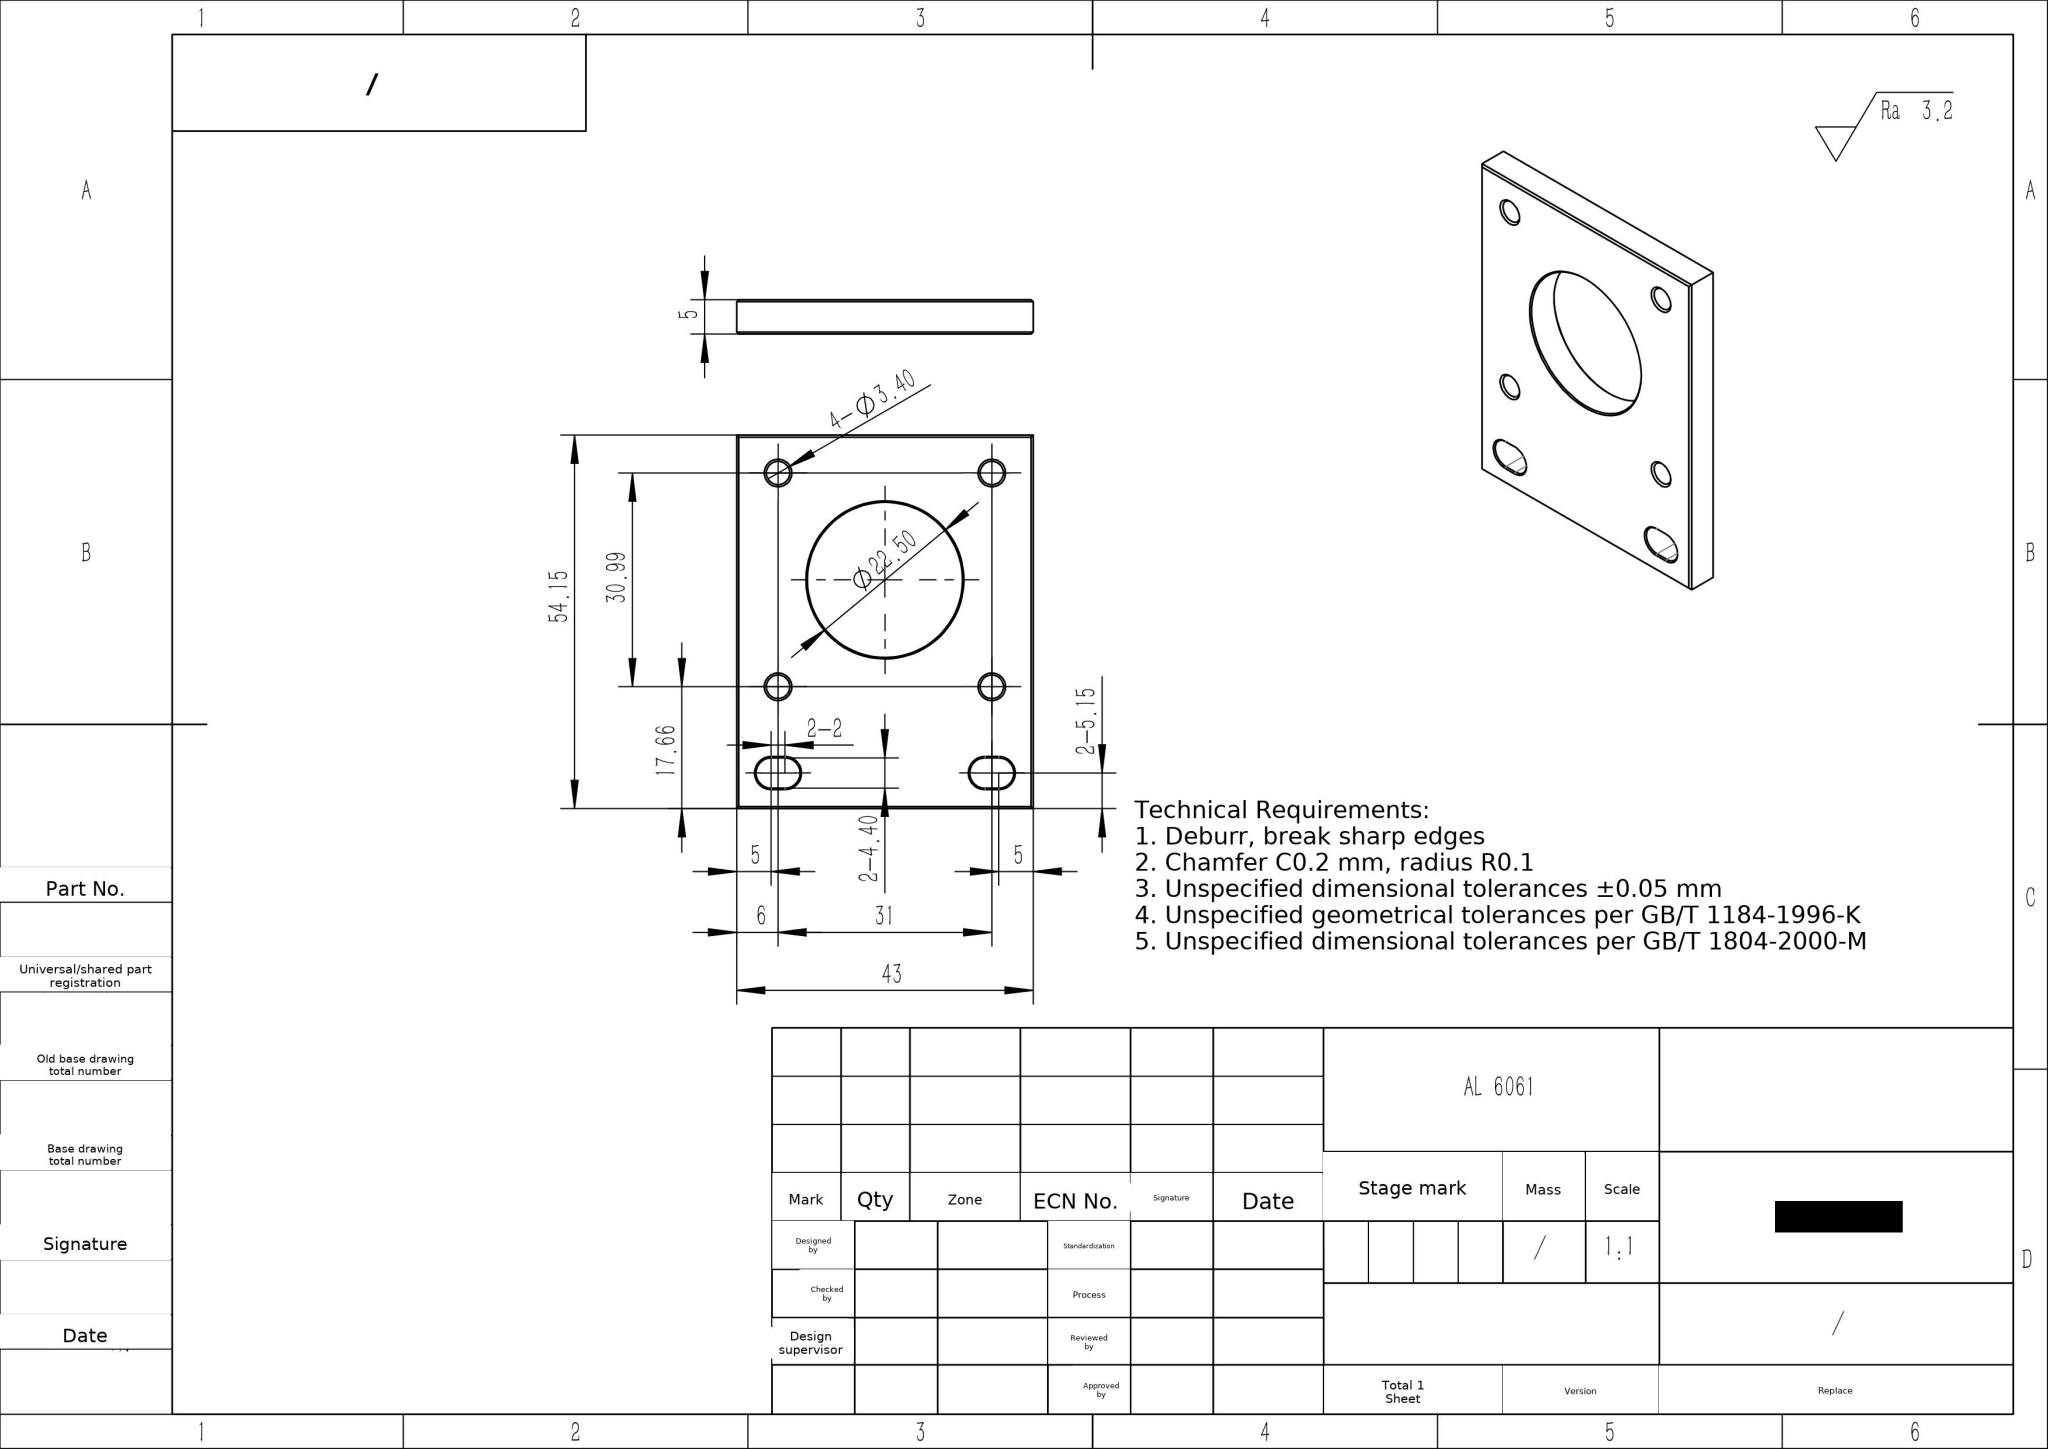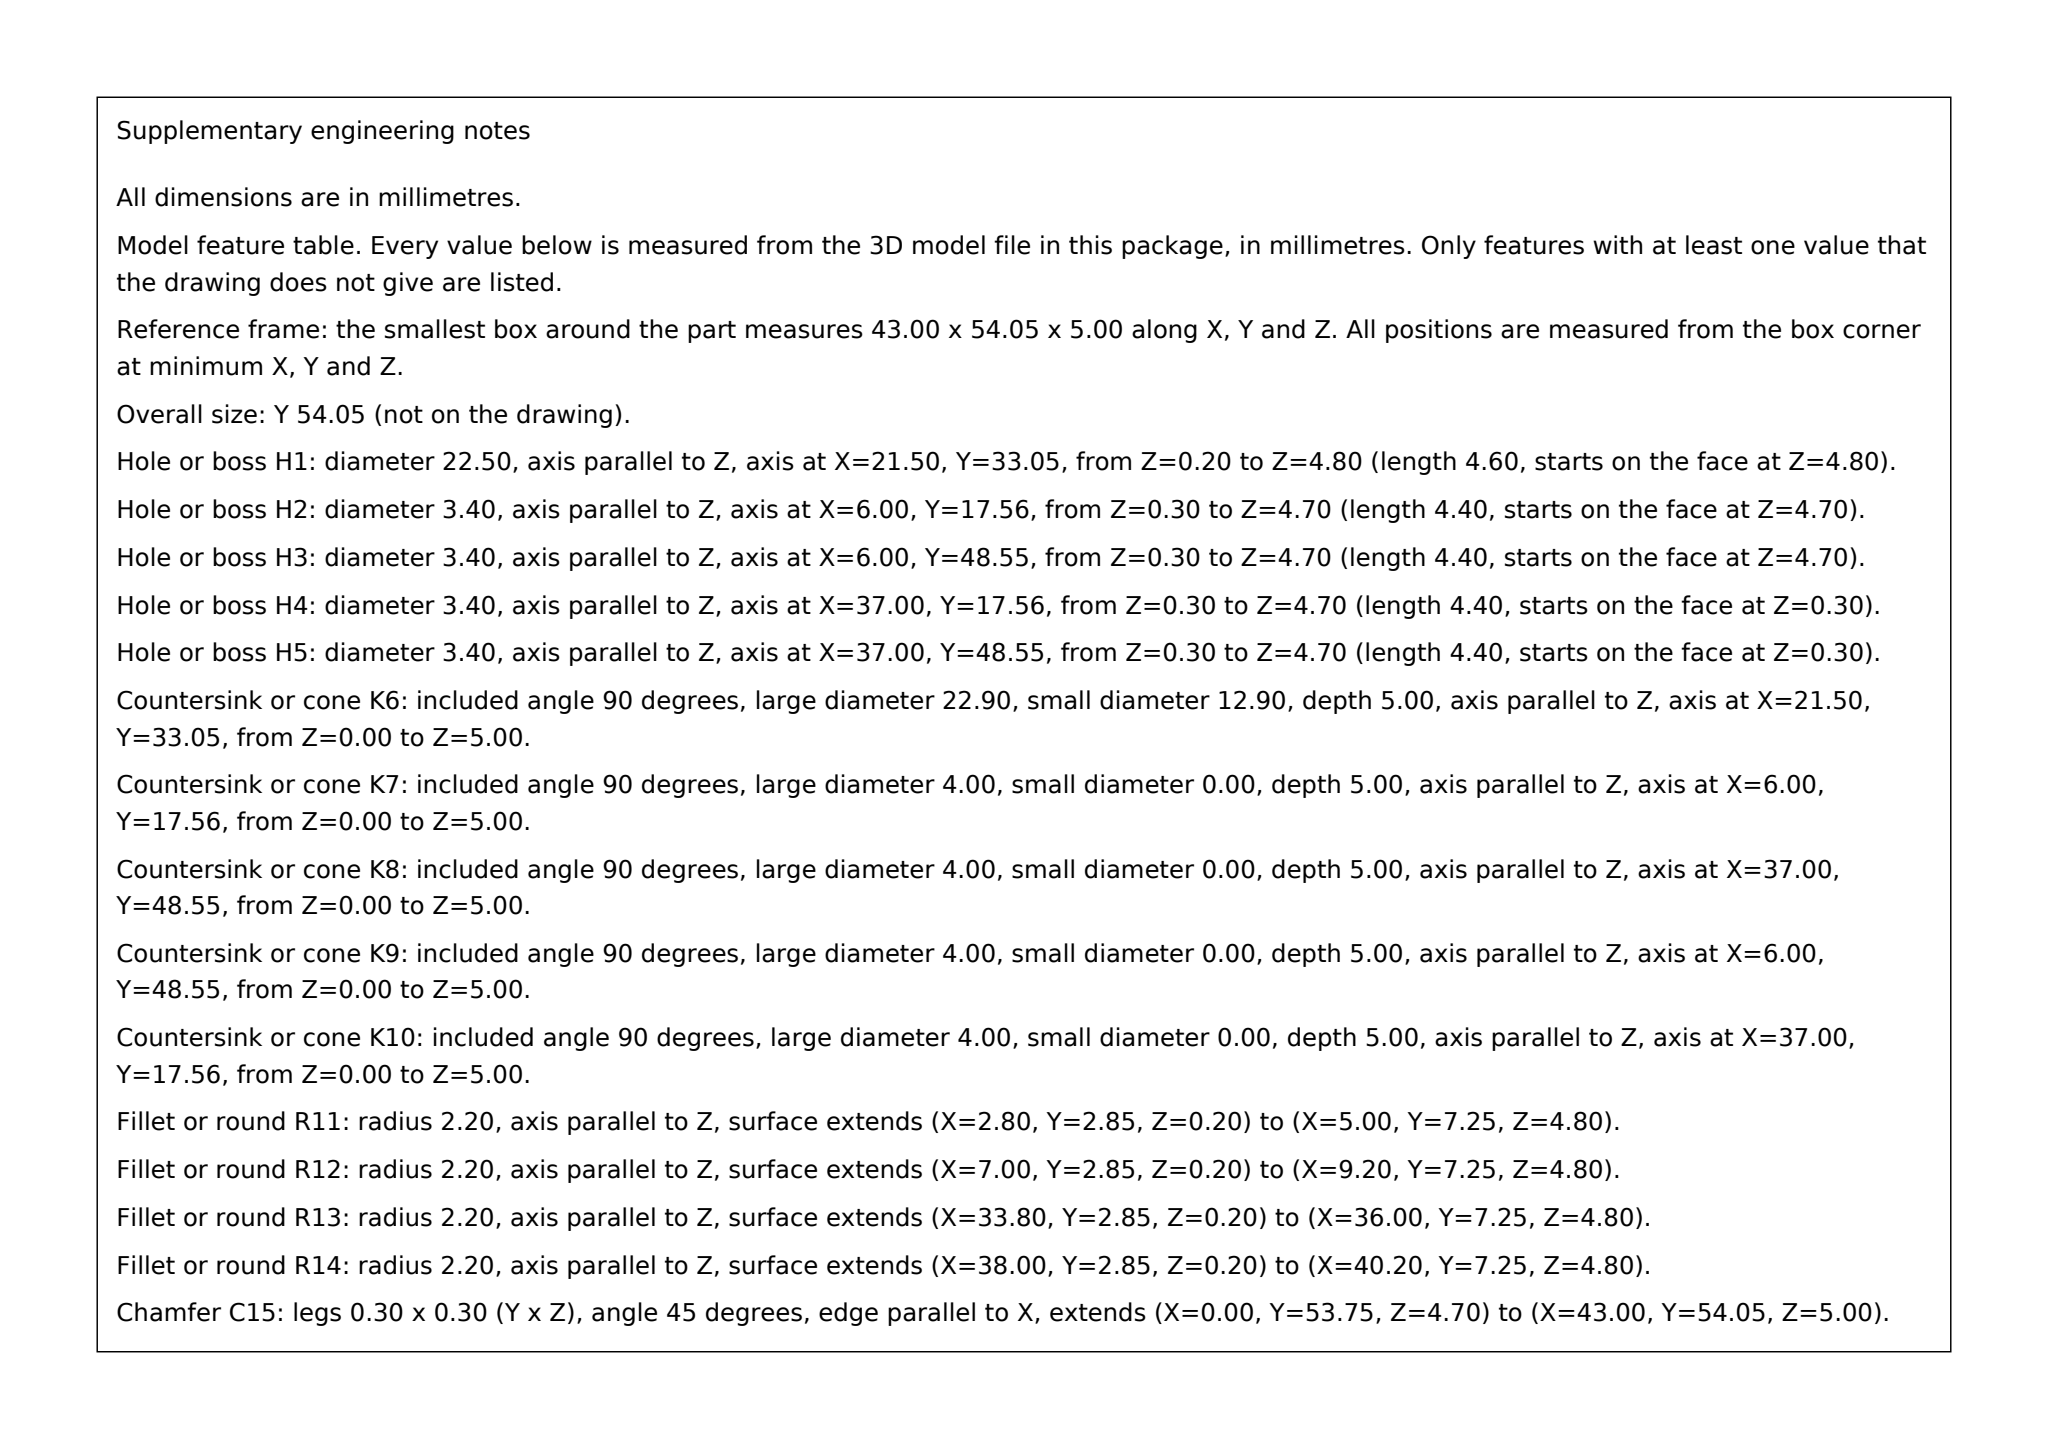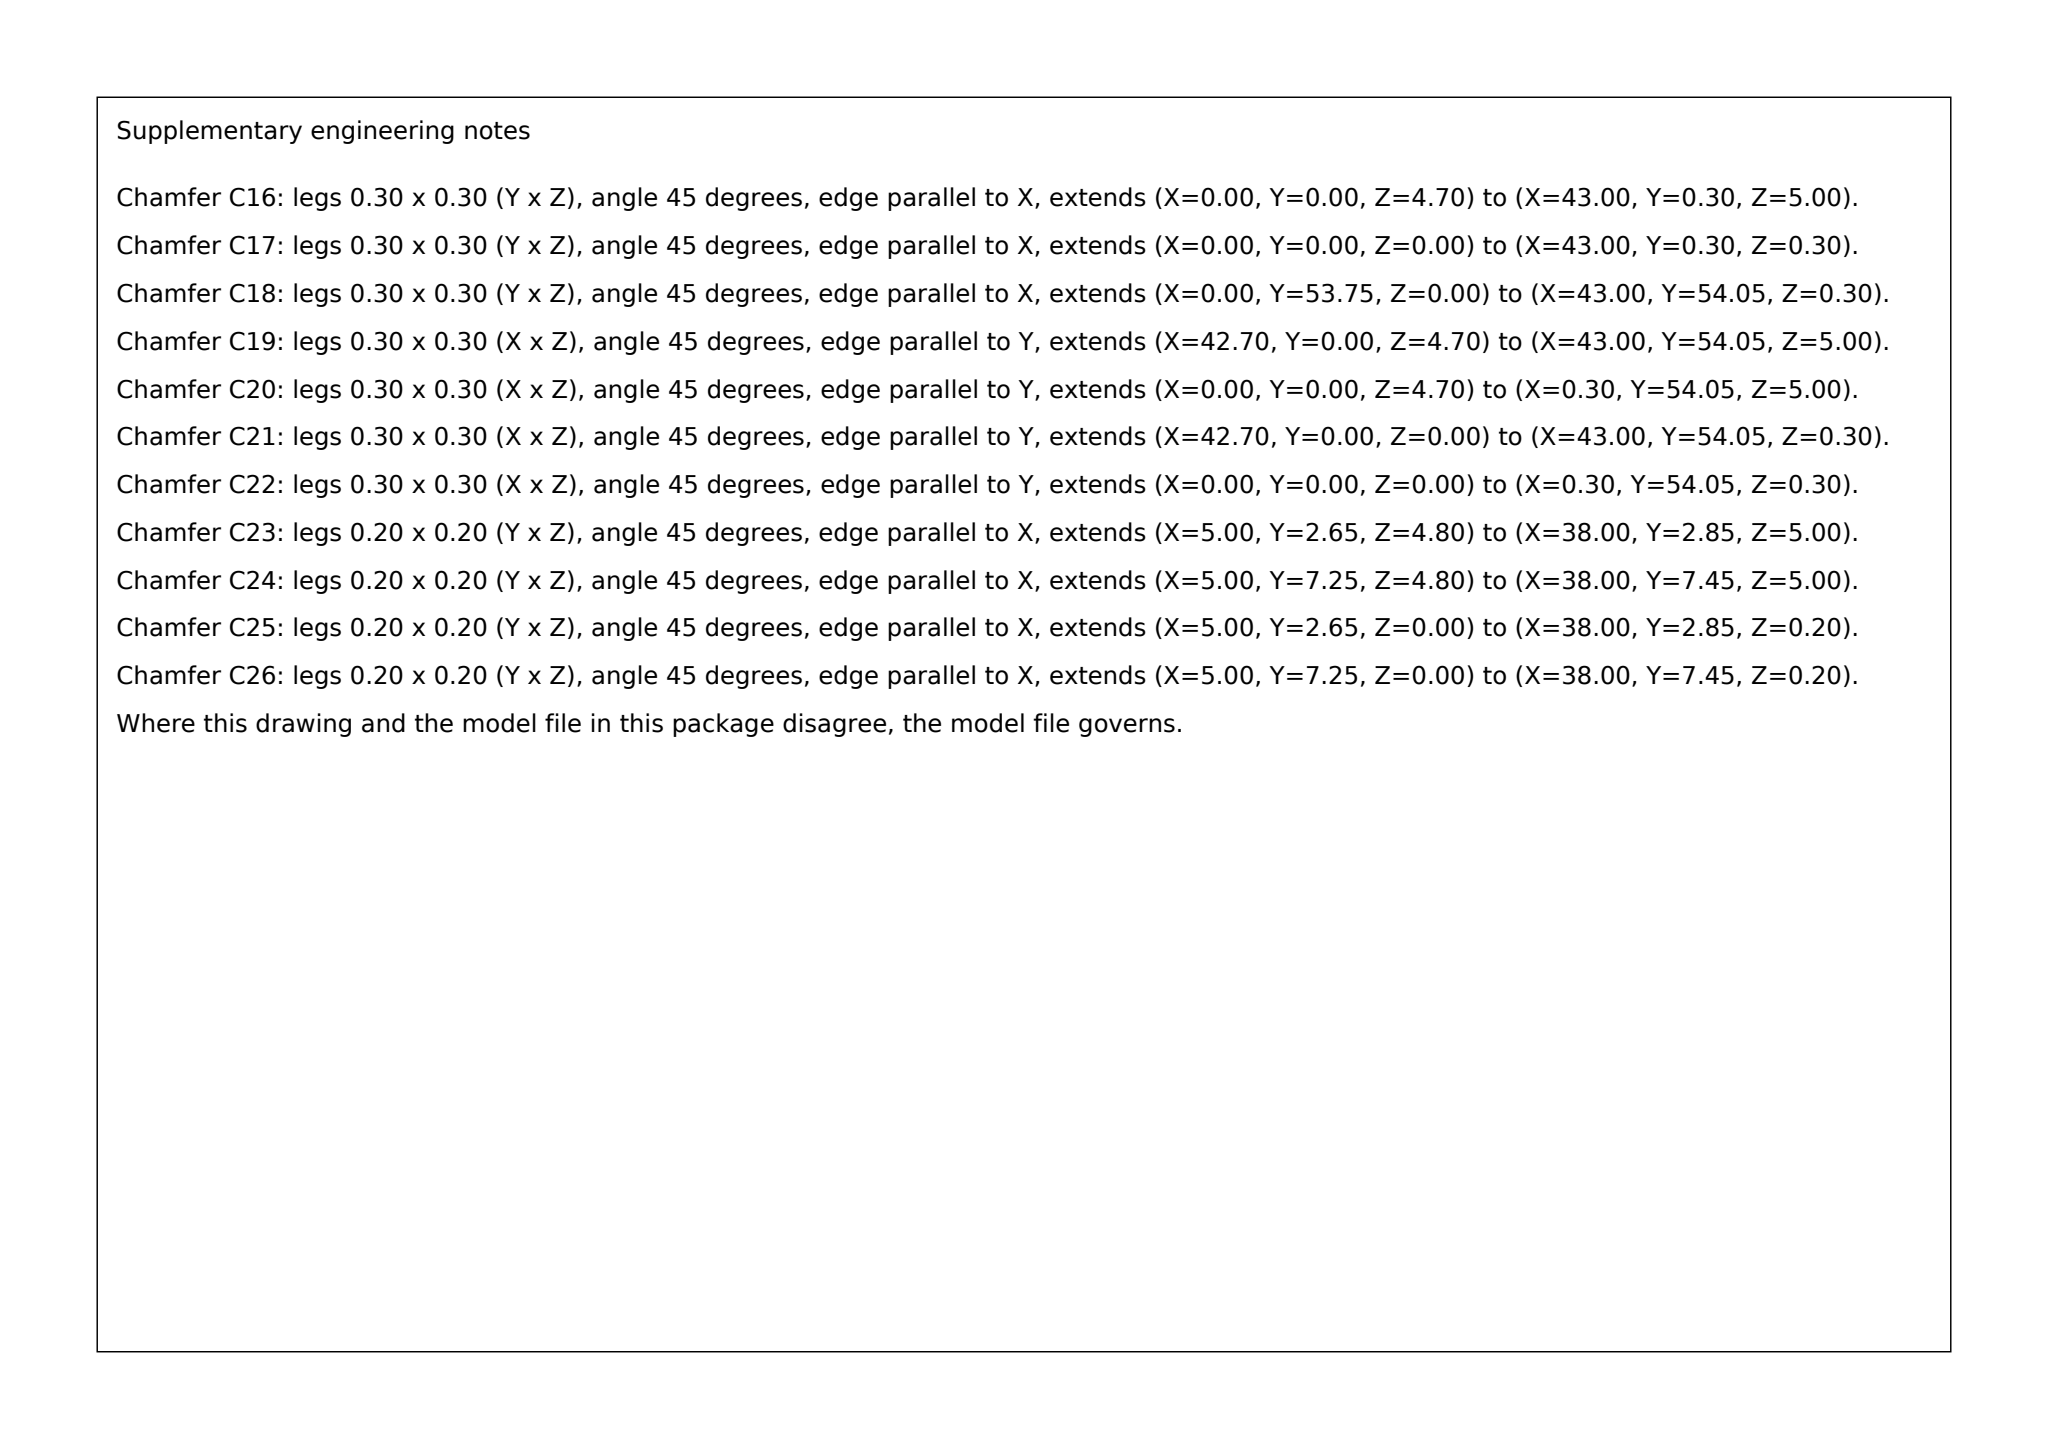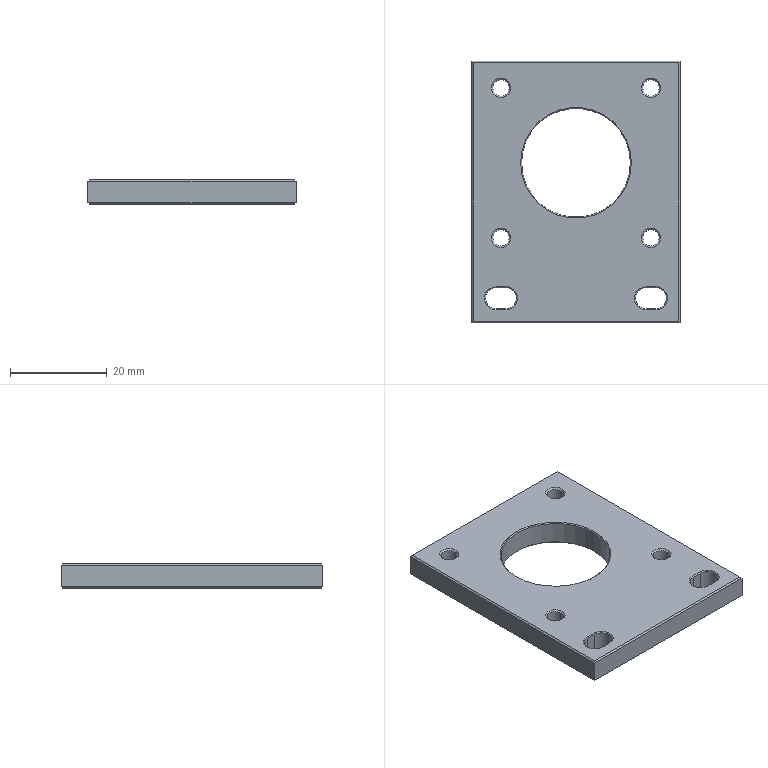Part | SolidWorks | mm | material AL 6061 | 1 solid | 74 faces | box 43 x 54.05 x 5 mm | volume 9185 mm3 | cone 32 | plane 26 | cylinder 16 | commonest cylinder face diameters 3.4 x8 4.4 x6 22.5 x2